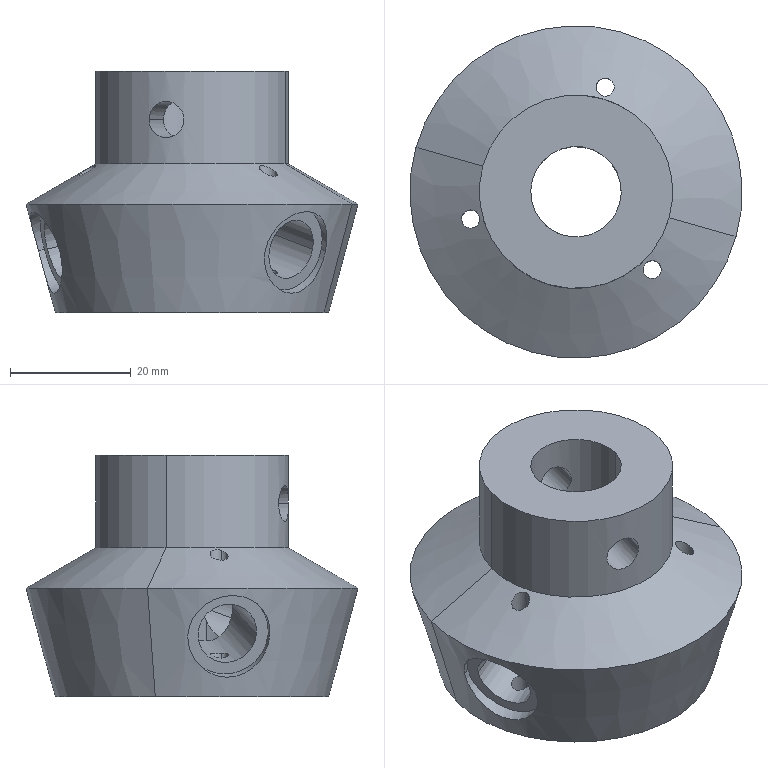Component | SolidWorks | Nut15InMulti-HandleNut-3 | 1 solid | 44 faces | volume 44343 mm3 | cylinder 34 | plane 6 | cone 4 | commonest cylinder face diameters 3 x12 10 x6 14 x6 6 x4 15 x2 18 x2 32 x2